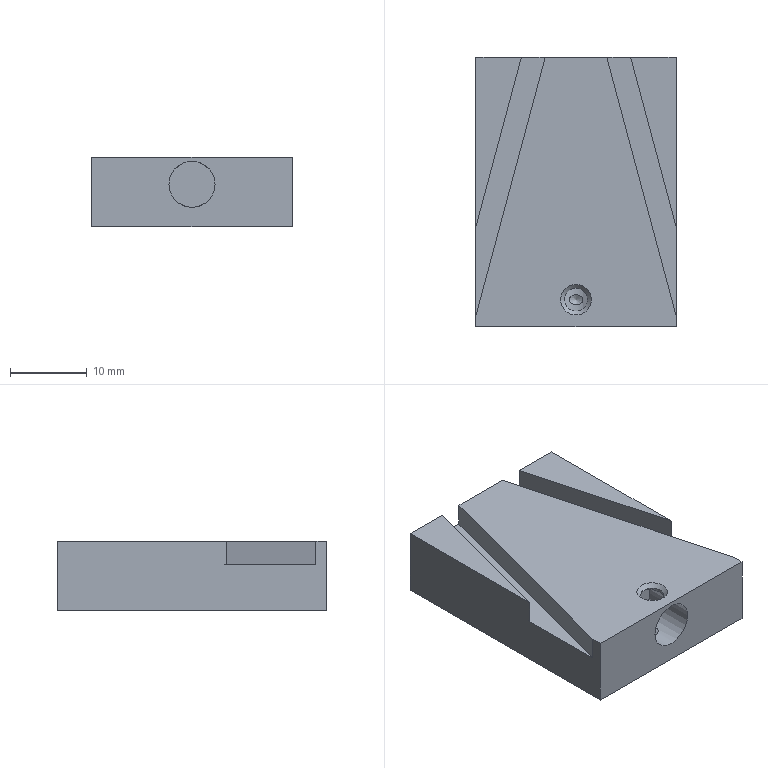Component | NX | SLIDER | 1 solid | 20 faces | volume 7468 mm3 | plane 15 | cylinder 3 | cone 2 | commonest cylinder face diameters 3 x2 6 x1